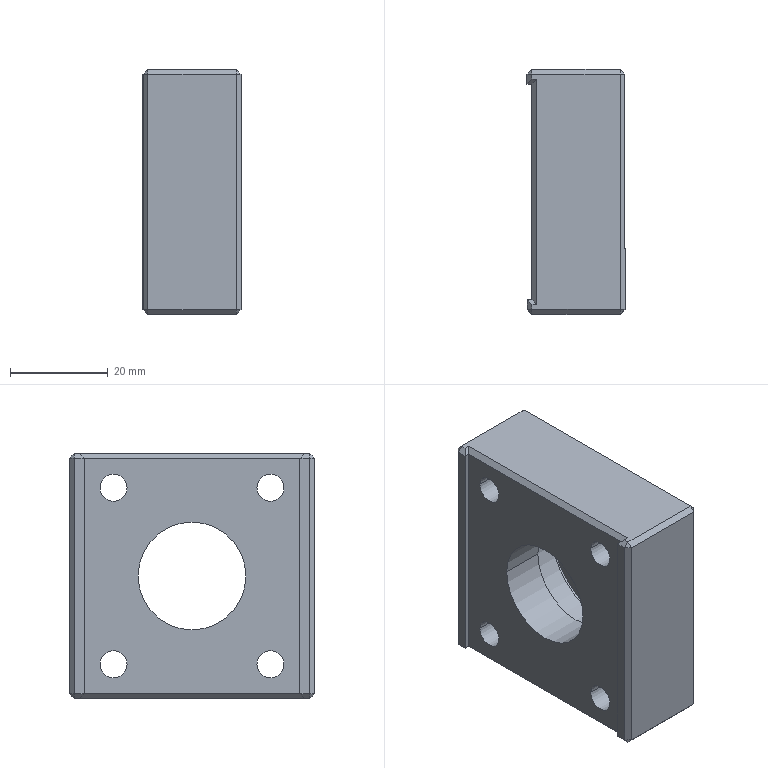Component | SolidWorks | SlidingPlate-1 | 1 solid | 69 faces | box 20.01 x 50 x 50 mm | volume 34785 mm3 | plane 45 | cylinder 24 | commonest cylinder face diameters 10 x8 5.5 x8 28 x4 31 x2 22 x2
build123d program:
from build123d import *

# Parameters (mm, degrees)
SKETCH1_W                                       = 50
SKETCH1_H                                       = 50
BOSS_EXTRUDE1_DEPTH                             = 20
M5_HEX_SOCKET_HEAD_CAP_SCREW_CBORE1_D           = 5.5
M5_HEX_SOCKET_HEAD_CAP_SCREW_CBORE1_CBORE_D     = 10
M5_HEX_SOCKET_HEAD_CAP_SCREW_CBORE1_CBORE_DEPTH = 5.4
SKETCH4_R                                       = 14
CUT_EXTRUDE1_DEPTH                              = 10
CUT_EXTRUDE2_REACH                              = 61.372
SKETCH5_W                                       = 44
SKETCH5_H                                       = 1.001
SKETCH6_R                                       = 11
CUT_EXTRUDE3_DEPTH                              = 12
CUT_EXTRUDE4_START                              = -3
SKETCH7_R                                       = 15.5
CUT_EXTRUDE4_DEPTH                              = 1.5
CHAMFER1_SIZE                                   = 1


with BuildPart() as part:
    # Sketch1 → Boss-Extrude1 (new body)
    with BuildSketch(Plane.XY):
        Rectangle(SKETCH1_W, SKETCH1_H)
    extrude(amount=BOSS_EXTRUDE1_DEPTH)

    # M5 Hex Socket Head Cap Screw CBORE1 (through all)
    with Locations(Plane.XY.offset(20)):
        with Locations((-16, 18), (16, 18), (-16, -18), (16, -18)):
            CounterBoreHole(M5_HEX_SOCKET_HEAD_CAP_SCREW_CBORE1_D / 2, M5_HEX_SOCKET_HEAD_CAP_SCREW_CBORE1_CBORE_D / 2, M5_HEX_SOCKET_HEAD_CAP_SCREW_CBORE1_CBORE_DEPTH)

    # Sketch4 → Cut-Extrude1 (cut)
    with BuildSketch(Plane.XY.offset(20)):
        Circle(SKETCH4_R)
    extrude(amount=-CUT_EXTRUDE1_DEPTH, mode=Mode.SUBTRACT)

    # Cut-Extrude2: up to this face of the body (flat: up to its plane)
    cut_extrude2_end = Plane(part.part.faces().sort_by_distance((0, 25, 10))[0])
    # Sketch5 → Cut-Extrude2 (cut, up to the picked face)
    with BuildSketch(Plane.XZ.offset(25), mode=Mode.PRIVATE) as cut_extrude2_sk1:
        with Locations((0, 0.5005)):
            Rectangle(SKETCH5_W, SKETCH5_H)
    cut_extrude2_tool1 = split(extrude(cut_extrude2_sk1.sketch, amount=-CUT_EXTRUDE2_REACH, mode=Mode.PRIVATE), bisect_by=cut_extrude2_end, keep=Keep.BOTH, mode=Mode.PRIVATE)
    add(cut_extrude2_tool1.solids().sort_by(Axis((0, -25, 0.5005), (0, 1, 0)))[0], mode=Mode.SUBTRACT)

    # Sketch6 → Cut-Extrude3 (cut)
    with BuildSketch(Plane(origin=(0, 0, 1.001), x_dir=(-1, 0, 0), z_dir=(0, 0, -1))):
        Circle(SKETCH6_R)
    extrude(amount=-CUT_EXTRUDE3_DEPTH, mode=Mode.SUBTRACT)

    # Sketch7 → Cut-Extrude4 (cut)
    with BuildSketch(Plane.XY.offset(20).offset(CUT_EXTRUDE4_START)):
        Circle(SKETCH7_R)
    extrude(amount=CUT_EXTRUDE4_DEPTH, mode=Mode.SUBTRACT)

    # Chamfer1
    chamfer1_edges = [part.edges().sort_by_distance(p)[0] for p in [
        (25, 0, 20),
        (0, 25, 20),
        (-25, 0, 20),
        (23.5, 25, 0),
        (25, 0, 0),
        (-23.5, 25, 0),
        (-23.5, -25, 0),
        (23.5, -25, 0),
        (-25, 0, 0),
        (-22, -25, 0.5005),
        (22, -25, 0.5005),
        (0, -25, 1.001),
        (-22, 25, 0.5005),
        (0, 25, 1.001),
        (22, 25, 0.5005),
        (0, -25, 20),
        (-25, 25, 10),
        (25, 25, 10),
        (25, -25, 10),
        (-25, -25, 10),
    ]]
    chamfer(chamfer1_edges, length=CHAMFER1_SIZE)


solid = part.part

# Placed as in the assembly
solid = solid.moved(Location((1531.163, 3833.695, 1079.241), (90, 90, 0)))